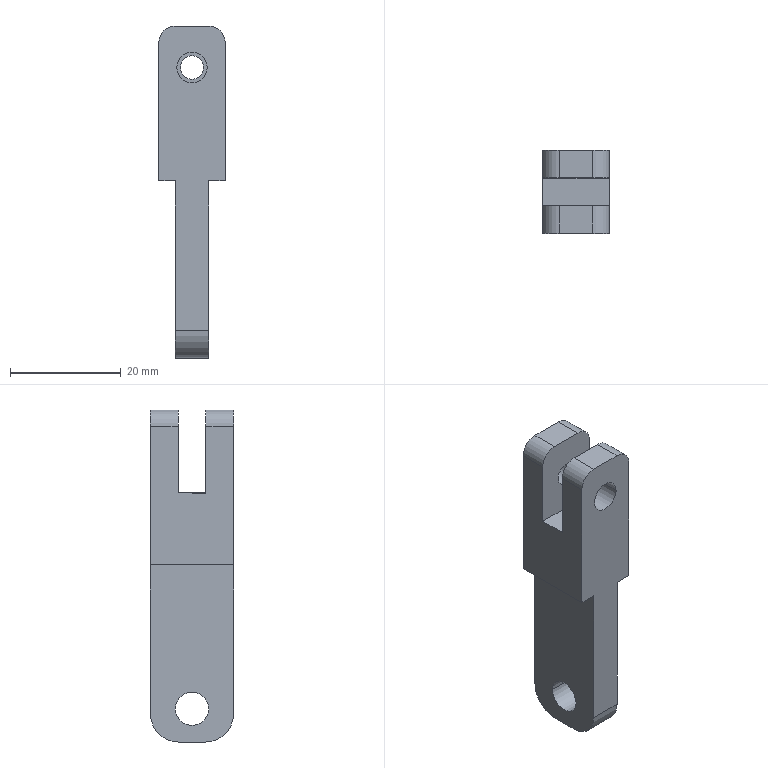Component | SolidWorks | ConnectingHinge1-2 | 1 solid | 26 faces | box 12 x 15 x 60 mm | volume 6559 mm3 | plane 14 | cylinder 12 | commonest cylinder face diameters 6 x6 4.2 x2 5.5 x2 10 x2
build123d program:
from build123d import *

# Parameters (mm, degrees)
SKETCH1_W           = 12
SKETCH1_H           = 60
BOSS_EXTRUDE1_DEPTH = 15
SKETCH2_W           = 5
SKETCH2_H           = 15
CUT_EXTRUDE1_DEPTH  = 64
CUT_EXTRUDE2_REACH  = 65
SKETCH3_R           = 2.75
M5_TAPPED_HOLE1_D   = 4.2
SKETCH6_R           = 3
CUT_EXTRUDE3_DEPTH  = 64
SKETCH7_W           = 3
SKETCH7_H           = 32
CUT_EXTRUDE4_DEPTH  = 64
FILLET1_R           = 5
FILLET2_R           = 3


with BuildPart() as part:
    # Sketch1 → Boss-Extrude1 (new body)
    with BuildSketch(Plane.XY):
        with Locations((6, 30)):
            Rectangle(SKETCH1_W, SKETCH1_H)
    extrude(amount=BOSS_EXTRUDE1_DEPTH)

    # Sketch2 → Cut-Extrude1 (cut, through all)
    with BuildSketch(Plane(origin=(12, 0, 0), x_dir=(0, 0, -1), z_dir=(1, 0, 0))):
        with Locations((-7.5, 7.5)):
            Rectangle(SKETCH2_W, SKETCH2_H)
    extrude(amount=-CUT_EXTRUDE1_DEPTH, mode=Mode.SUBTRACT)

    # Sketch3 → Cut-Extrude2 (cut, up to next)
    with BuildSketch(Plane(origin=(0, 0, 0), x_dir=(-1, 0, 0), z_dir=(0, 0, -1)), mode=Mode.PRIVATE) as cut_extrude2_sk1:
        with Locations((-6, 7.5)):
            Circle(SKETCH3_R)
    cut_extrude2_tool1 = extrude(cut_extrude2_sk1.sketch, amount=-CUT_EXTRUDE2_REACH, mode=Mode.PRIVATE) & part.part
    add(cut_extrude2_tool1.solids().sort_by_distance((6, 7.5, 0))[0], mode=Mode.SUBTRACT)

    # M5 Tapped Hole1 (through all)
    with Locations(Plane(origin=(6, 7.5, 15), x_dir=(1, 0, 0), z_dir=(0, 0, 1))):
        with Locations((0, 0)):
            Hole(M5_TAPPED_HOLE1_D / 2)

    # Sketch6 → Cut-Extrude3 (cut, through all)
    with BuildSketch(Plane.ZY):
        with Locations((7.5, 54)):
            Circle(SKETCH6_R)
    extrude(amount=-CUT_EXTRUDE3_DEPTH, mode=Mode.SUBTRACT)

    # Sketch7 → Cut-Extrude4 (cut, through all)
    with BuildSketch(Plane.XY.offset(15)):
        with Locations((1.5, 44)):
            Rectangle(SKETCH7_W, SKETCH7_H)
        with Locations((10.5, 44)):
            Rectangle(SKETCH7_W, SKETCH7_H)
    extrude(amount=-CUT_EXTRUDE4_DEPTH, mode=Mode.SUBTRACT)

    # Fillet1
    fillet1_edges = [part.edges().sort_by_distance(p)[0] for p in [
        (6, 60, 0),
        (6, 60, 15),
    ]]
    fillet(fillet1_edges, radius=FILLET1_R)

    # Fillet2
    fillet2_edges = [part.edges().sort_by_distance(p)[0] for p in [
        (12, 0, 2.5),
        (0, 0, 2.5),
        (12, 0, 12.5),
        (0, 0, 12.5),
    ]]
    fillet(fillet2_edges, radius=FILLET2_R)


solid = part.part

# Placed as in the assembly
solid = solid.moved(Location((-16, -226.728, 142.5), (-90, 0, 0)))
STEP:
#1=COLOUR_RGB('',0.7922,0.8196,0.9333);
#2=FILL_AREA_STYLE_COLOUR('',#1);
#3=FILL_AREA_STYLE('',(#2));
#4=SURFACE_STYLE_FILL_AREA(#3);
#5=SURFACE_SIDE_STYLE('',(#4));
#6=SURFACE_STYLE_USAGE(.BOTH.,#5);
#7=PRESENTATION_STYLE_ASSIGNMENT((#6));
#8=CARTESIAN_POINT('',(-0.2756,-8.513,3.484));
#9=VERTEX_POINT('',#8);
#10=CARTESIAN_POINT('',(-0.2756,-8.749,3.484));
#11=VERTEX_POINT('',#10);
#12=CARTESIAN_POINT('',(-0.2756,-8.631,3.484));
#13=DIRECTION('',(1.,0.,0.));
#14=DIRECTION('',(-0.,0.,1.));
#15=AXIS2_PLACEMENT_3D('',#12,#13,#14);
#16=CIRCLE('',#15,0.1181);
#17=EDGE_CURVE('',#9,#11,#16,.T.);
#18=ORIENTED_EDGE('',*,*,#17,.T.);
#19=CARTESIAN_POINT('',(-0.5118,-8.749,3.484));
#20=VERTEX_POINT('',#19);
#21=CARTESIAN_POINT('',(-0.1575,-8.749,3.484));
#22=DIRECTION('',(-1.,-0.,-0.));
#23=VECTOR('',#22,39.37);
#24=LINE('',#21,#23);
#25=EDGE_CURVE('',#11,#20,#24,.T.);
#26=ORIENTED_EDGE('',*,*,#25,.T.);
#27=CARTESIAN_POINT('',(-0.5118,-8.513,3.484));
#28=VERTEX_POINT('',#27);
#29=CARTESIAN_POINT('',(-0.5118,-8.631,3.484));
#30=DIRECTION('',(-1.,-0.,-0.));
#31=DIRECTION('',(0.,0.,-1.));
#32=AXIS2_PLACEMENT_3D('',#29,#30,#31);
#33=CIRCLE('',#32,0.1181);
#34=EDGE_CURVE('',#20,#28,#33,.T.);
#35=ORIENTED_EDGE('',*,*,#34,.T.);
#36=CARTESIAN_POINT('',(-0.1575,-8.513,3.484));
#37=DIRECTION('',(-1.,-0.,-0.));
#38=VECTOR('',#37,39.37);
#39=LINE('',#36,#38);
#40=EDGE_CURVE('',#9,#28,#39,.T.);
#41=ORIENTED_EDGE('',*,*,#40,.F.);
#42=EDGE_LOOP('',(#18,#26,#35,#41));
#43=FACE_OUTER_BOUND('',#42,.T.);
#44=CARTESIAN_POINT('',(-0.1575,-8.631,3.484));
#45=DIRECTION('',(-1.,-0.,-0.));
#46=DIRECTION('',(-0.,1.,0.));
#47=AXIS2_PLACEMENT_3D('',#44,#45,#46);
#48=CYLINDRICAL_SURFACE('',#47,0.1181);
#49=ADVANCED_FACE('',(#43),#48,.F.);
#50=CARTESIAN_POINT('',(-0.4764,-8.533,5.315));
#51=VERTEX_POINT('',#50);
#52=CARTESIAN_POINT('',(-0.311,-8.533,5.315));
#53=VERTEX_POINT('',#52);
#54=CARTESIAN_POINT('',(-0.3937,-8.533,5.315));
#55=DIRECTION('',(-0.,1.,0.));
#56=DIRECTION('',(-0.,0.,1.));
#57=AXIS2_PLACEMENT_3D('',#54,#55,#56);
#58=CIRCLE('',#57,0.08268);
#59=EDGE_CURVE('',#51,#53,#58,.T.);
#60=ORIENTED_EDGE('',*,*,#59,.F.);
#61=CARTESIAN_POINT('',(-0.4764,-8.336,5.315));
#62=VERTEX_POINT('',#61);
#63=CARTESIAN_POINT('',(-0.4764,-8.336,5.315));
#64=DIRECTION('',(-0.,1.,0.));
#65=VECTOR('',#64,39.37);
#66=LINE('',#63,#65);
#67=EDGE_CURVE('',#51,#62,#66,.T.);
#68=ORIENTED_EDGE('',*,*,#67,.T.);
#69=CARTESIAN_POINT('',(-0.311,-8.336,5.315));
#70=VERTEX_POINT('',#69);
#71=CARTESIAN_POINT('',(-0.3937,-8.336,5.315));
#72=DIRECTION('',(-0.,1.,0.));
#73=DIRECTION('',(1.,0.,0.));
#74=AXIS2_PLACEMENT_3D('',#71,#72,#73);
#75=CIRCLE('',#74,0.08268);
#76=EDGE_CURVE('',#62,#70,#75,.T.);
#77=ORIENTED_EDGE('',*,*,#76,.T.);
#78=CARTESIAN_POINT('',(-0.311,-8.336,5.315));
#79=DIRECTION('',(-0.,1.,0.));
#80=VECTOR('',#79,39.37);
#81=LINE('',#78,#80);
#82=EDGE_CURVE('',#53,#70,#81,.T.);
#83=ORIENTED_EDGE('',*,*,#82,.F.);
#84=EDGE_LOOP('',(#60,#68,#77,#83));
#85=FACE_OUTER_BOUND('',#84,.T.);
#86=CARTESIAN_POINT('',(-0.3937,-8.336,5.315));
#87=DIRECTION('',(-0.,1.,0.));
#88=DIRECTION('',(1.,0.,0.));
#89=AXIS2_PLACEMENT_3D('',#86,#87,#88);
#90=CYLINDRICAL_SURFACE('',#89,0.08268);
#91=ADVANCED_FACE('',(#85),#90,.F.);
#92=CARTESIAN_POINT('',(-0.502,-8.729,5.315));
#93=VERTEX_POINT('',#92);
#94=CARTESIAN_POINT('',(-0.2854,-8.729,5.315));
#95=VERTEX_POINT('',#94);
#96=CARTESIAN_POINT('',(-0.3937,-8.729,5.315));
#97=DIRECTION('',(-0.,1.,0.));
#98=DIRECTION('',(0.,0.,-1.));
#99=AXIS2_PLACEMENT_3D('',#96,#97,#98);
#100=CIRCLE('',#99,0.1083);
#101=EDGE_CURVE('',#93,#95,#100,.T.);
#102=ORIENTED_EDGE('',*,*,#101,.T.);
#103=CARTESIAN_POINT('',(-0.2854,-8.926,5.315));
#104=VERTEX_POINT('',#103);
#105=CARTESIAN_POINT('',(-0.2854,-8.336,5.315));
#106=DIRECTION('',(0.,-1.,-0.));
#107=VECTOR('',#106,39.37);
#108=LINE('',#105,#107);
#109=EDGE_CURVE('',#95,#104,#108,.T.);
#110=ORIENTED_EDGE('',*,*,#109,.T.);
#111=CARTESIAN_POINT('',(-0.502,-8.926,5.315));
#112=VERTEX_POINT('',#111);
#113=CARTESIAN_POINT('',(-0.3937,-8.926,5.315));
#114=DIRECTION('',(0.,-1.,-0.));
#115=DIRECTION('',(-1.,0.,0.));
#116=AXIS2_PLACEMENT_3D('',#113,#114,#115);
#117=CIRCLE('',#116,0.1083);
#118=EDGE_CURVE('',#104,#112,#117,.T.);
#119=ORIENTED_EDGE('',*,*,#118,.T.);
#120=CARTESIAN_POINT('',(-0.502,-8.336,5.315));
#121=DIRECTION('',(0.,-1.,-0.));
#122=VECTOR('',#121,39.37);
#123=LINE('',#120,#122);
#124=EDGE_CURVE('',#93,#112,#123,.T.);
#125=ORIENTED_EDGE('',*,*,#124,.F.);
#126=EDGE_LOOP('',(#102,#110,#119,#125));
#127=FACE_OUTER_BOUND('',#126,.T.);
#128=CARTESIAN_POINT('',(-0.3937,-8.336,5.315));
#129=DIRECTION('',(0.,-1.,-0.));
#130=DIRECTION('',(-1.,0.,0.));
#131=AXIS2_PLACEMENT_3D('',#128,#129,#130);
#132=CYLINDRICAL_SURFACE('',#131,0.1083);
#133=ADVANCED_FACE('',(#127),#132,.F.);
#134=CARTESIAN_POINT('',(-0.6299,-8.336,4.508));
#135=VERTEX_POINT('',#134);
#136=CARTESIAN_POINT('',(-0.6299,-8.336,5.492));
#137=VERTEX_POINT('',#136);
#138=CARTESIAN_POINT('',(-0.6299,-8.336,5.61));
#139=DIRECTION('',(-0.,-0.,1.));
#140=VECTOR('',#139,39.37);
#141=LINE('',#138,#140);
#142=EDGE_CURVE('',#135,#137,#141,.T.);
#143=ORIENTED_EDGE('',*,*,#142,.T.);
#144=CARTESIAN_POINT('',(-0.5118,-8.336,5.61));
#145=VERTEX_POINT('',#144);
#146=CARTESIAN_POINT('',(-0.5118,-8.336,5.492));
#147=DIRECTION('',(-0.,1.,0.));
#148=DIRECTION('',(-1.,0.,0.));
#149=AXIS2_PLACEMENT_3D('',#146,#147,#148);
#150=CIRCLE('',#149,0.1181);
#151=EDGE_CURVE('',#137,#145,#150,.T.);
#152=ORIENTED_EDGE('',*,*,#151,.T.);
#153=CARTESIAN_POINT('',(-0.2756,-8.336,5.61));
#154=VERTEX_POINT('',#153);
#155=CARTESIAN_POINT('',(-0.6299,-8.336,5.61));
#156=DIRECTION('',(1.,0.,0.));
#157=VECTOR('',#156,39.37);
#158=LINE('',#155,#157);
#159=EDGE_CURVE('',#145,#154,#158,.T.);
#160=ORIENTED_EDGE('',*,*,#159,.T.);
#161=CARTESIAN_POINT('',(-0.1575,-8.336,5.492));
#162=VERTEX_POINT('',#161);
#163=CARTESIAN_POINT('',(-0.2756,-8.336,5.492));
#164=DIRECTION('',(-0.,1.,0.));
#165=DIRECTION('',(-1.,0.,0.));
#166=AXIS2_PLACEMENT_3D('',#163,#164,#165);
#167=CIRCLE('',#166,0.1181);
#168=EDGE_CURVE('',#154,#162,#167,.T.);
#169=ORIENTED_EDGE('',*,*,#168,.T.);
#170=CARTESIAN_POINT('',(-0.1575,-8.336,4.508));
#171=VERTEX_POINT('',#170);
#172=CARTESIAN_POINT('',(-0.1575,-8.336,5.61));
#173=DIRECTION('',(0.,0.,-1.));
#174=VECTOR('',#173,39.37);
#175=LINE('',#172,#174);
#176=EDGE_CURVE('',#162,#171,#175,.T.);
#177=ORIENTED_EDGE('',*,*,#176,.T.);
#178=CARTESIAN_POINT('',(-0.2756,-8.336,4.508));
#179=VERTEX_POINT('',#178);
#180=CARTESIAN_POINT('',(-0.1575,-8.336,4.508));
#181=DIRECTION('',(1.,0.,0.));
#182=VECTOR('',#181,39.37);
#183=LINE('',#180,#182);
#184=EDGE_CURVE('',#179,#171,#183,.T.);
#185=ORIENTED_EDGE('',*,*,#184,.F.);
#186=CARTESIAN_POINT('',(-0.2756,-8.336,3.445));
#187=VERTEX_POINT('',#186);
#188=CARTESIAN_POINT('',(-0.2756,-8.336,3.248));
#189=DIRECTION('',(-0.,-0.,1.));
#190=VECTOR('',#189,39.37);
#191=LINE('',#188,#190);
#192=EDGE_CURVE('',#187,#179,#191,.T.);
#193=ORIENTED_EDGE('',*,*,#192,.F.);
#194=CARTESIAN_POINT('',(-0.5118,-8.336,3.445));
#195=VERTEX_POINT('',#194);
#196=CARTESIAN_POINT('',(-0.6299,-8.336,3.445));
#197=DIRECTION('',(-1.,-0.,-0.));
#198=VECTOR('',#197,39.37);
#199=LINE('',#196,#198);
#200=EDGE_CURVE('',#187,#195,#199,.T.);
#201=ORIENTED_EDGE('',*,*,#200,.T.);
#202=CARTESIAN_POINT('',(-0.5118,-8.336,4.508));
#203=VERTEX_POINT('',#202);
#204=CARTESIAN_POINT('',(-0.5118,-8.336,3.248));
#205=DIRECTION('',(0.,0.,-1.));
#206=VECTOR('',#205,39.37);
#207=LINE('',#204,#206);
#208=EDGE_CURVE('',#203,#195,#207,.T.);
#209=ORIENTED_EDGE('',*,*,#208,.F.);
#210=CARTESIAN_POINT('',(-0.6299,-8.336,4.508));
#211=DIRECTION('',(1.,0.,0.));
#212=VECTOR('',#211,39.37);
#213=LINE('',#210,#212);
#214=EDGE_CURVE('',#135,#203,#213,.T.);
#215=ORIENTED_EDGE('',*,*,#214,.F.);
#216=EDGE_LOOP('',(#143,#152,#160,#169,#177,#185,#193,#201,#209,#215));
#217=FACE_OUTER_BOUND('',#216,.T.);
#218=CARTESIAN_POINT('',(-0.3937,-8.336,5.315));
#219=DIRECTION('',(-0.,1.,0.));
#220=DIRECTION('',(1.,0.,0.));
#221=AXIS2_PLACEMENT_3D('',#218,#219,#220);
#222=CIRCLE('',#221,0.08268);
#223=EDGE_CURVE('',#70,#62,#222,.T.);
#224=ORIENTED_EDGE('',*,*,#223,.F.);
#225=ORIENTED_EDGE('',*,*,#76,.F.);
#226=EDGE_LOOP('',(#224,#225));
#227=FACE_BOUND('',#226,.T.);
#228=CARTESIAN_POINT('',(-0.6299,-8.336,5.61));
#229=DIRECTION('',(0.,-1.,-0.));
#230=DIRECTION('',(-1.,-0.,-0.));
#231=AXIS2_PLACEMENT_3D('',#228,#229,#230);
#232=PLANE('',#231);
#233=ADVANCED_FACE('',(#217,#227),#232,.F.);
#234=ORIENTED_EDGE('',*,*,#159,.F.);
#235=CARTESIAN_POINT('',(-0.5118,-8.533,5.61));
#236=VERTEX_POINT('',#235);
#237=CARTESIAN_POINT('',(-0.5118,-8.336,5.61));
#238=DIRECTION('',(0.,-1.,-0.));
#239=VECTOR('',#238,39.37);
#240=LINE('',#237,#239);
#241=EDGE_CURVE('',#145,#236,#240,.T.);
#242=ORIENTED_EDGE('',*,*,#241,.T.);
#243=CARTESIAN_POINT('',(-0.2756,-8.533,5.61));
#244=VERTEX_POINT('',#243);
#245=CARTESIAN_POINT('',(-0.6299,-8.533,5.61));
#246=DIRECTION('',(1.,0.,0.));
#247=VECTOR('',#246,39.37);
#248=LINE('',#245,#247);
#249=EDGE_CURVE('',#236,#244,#248,.T.);
#250=ORIENTED_EDGE('',*,*,#249,.T.);
#251=CARTESIAN_POINT('',(-0.2756,-8.336,5.61));
#252=DIRECTION('',(-0.,1.,0.));
#253=VECTOR('',#252,39.37);
#254=LINE('',#251,#253);
#255=EDGE_CURVE('',#244,#154,#254,.T.);
#256=ORIENTED_EDGE('',*,*,#255,.T.);
#257=EDGE_LOOP('',(#234,#242,#250,#256));
#258=FACE_OUTER_BOUND('',#257,.T.);
#259=CARTESIAN_POINT('',(-0.6299,-8.336,5.61));
#260=DIRECTION('',(0.,0.,-1.));
#261=DIRECTION('',(-0.,1.,0.));
#262=AXIS2_PLACEMENT_3D('',#259,#260,#261);
#263=PLANE('',#262);
#264=ADVANCED_FACE('',(#258),#263,.F.);
#265=CARTESIAN_POINT('',(-0.6299,-8.533,5.02));
#266=VERTEX_POINT('',#265);
#267=CARTESIAN_POINT('',(-0.6299,-8.533,5.492));
#268=VERTEX_POINT('',#267);
#269=CARTESIAN_POINT('',(-0.6299,-8.533,5.02));
#270=DIRECTION('',(-0.,-0.,1.));
#271=VECTOR('',#270,39.37);
#272=LINE('',#269,#271);
#273=EDGE_CURVE('',#266,#268,#272,.T.);
#274=ORIENTED_EDGE('',*,*,#273,.T.);
#275=CARTESIAN_POINT('',(-0.6299,-8.336,5.492));
#276=DIRECTION('',(-0.,1.,0.));
#277=VECTOR('',#276,39.37);
#278=LINE('',#275,#277);
#279=EDGE_CURVE('',#268,#137,#278,.T.);
#280=ORIENTED_EDGE('',*,*,#279,.T.);
#281=ORIENTED_EDGE('',*,*,#142,.F.);
#282=CARTESIAN_POINT('',(-0.6299,-8.926,4.508));
#283=VERTEX_POINT('',#282);
#284=CARTESIAN_POINT('',(-0.6299,-8.926,4.508));
#285=DIRECTION('',(-0.,1.,0.));
#286=VECTOR('',#285,39.37);
#287=LINE('',#284,#286);
#288=EDGE_CURVE('',#283,#135,#287,.T.);
#289=ORIENTED_EDGE('',*,*,#288,.F.);
#290=CARTESIAN_POINT('',(-0.6299,-8.926,5.492));
#291=VERTEX_POINT('',#290);
#292=CARTESIAN_POINT('',(-0.6299,-8.926,5.61));
#293=DIRECTION('',(-0.,-0.,1.));
#294=VECTOR('',#293,39.37);
#295=LINE('',#292,#294);
#296=EDGE_CURVE('',#283,#291,#295,.T.);
#297=ORIENTED_EDGE('',*,*,#296,.T.);
#298=CARTESIAN_POINT('',(-0.6299,-8.729,5.492));
#299=VERTEX_POINT('',#298);
#300=CARTESIAN_POINT('',(-0.6299,-8.336,5.492));
#301=DIRECTION('',(-0.,1.,0.));
#302=VECTOR('',#301,39.37);
#303=LINE('',#300,#302);
#304=EDGE_CURVE('',#291,#299,#303,.T.);
#305=ORIENTED_EDGE('',*,*,#304,.T.);
#306=CARTESIAN_POINT('',(-0.6299,-8.729,5.02));
#307=VERTEX_POINT('',#306);
#308=CARTESIAN_POINT('',(-0.6299,-8.729,5.02));
#309=DIRECTION('',(0.,0.,-1.));
#310=VECTOR('',#309,39.37);
#311=LINE('',#308,#310);
#312=EDGE_CURVE('',#299,#307,#311,.T.);
#313=ORIENTED_EDGE('',*,*,#312,.T.);
#314=CARTESIAN_POINT('',(-0.6299,-8.533,5.02));
#315=DIRECTION('',(-0.,1.,0.));
#316=VECTOR('',#315,39.37);
#317=LINE('',#314,#316);
#318=EDGE_CURVE('',#307,#266,#317,.T.);
#319=ORIENTED_EDGE('',*,*,#318,.T.);
#320=EDGE_LOOP('',(#274,#280,#281,#289,#297,#305,#313,#319));
#321=FACE_OUTER_BOUND('',#320,.T.);
#322=CARTESIAN_POINT('',(-0.6299,-8.336,5.61));
#323=DIRECTION('',(1.,0.,0.));
#324=DIRECTION('',(0.,-1.,-0.));
#325=AXIS2_PLACEMENT_3D('',#322,#323,#324);
#326=PLANE('',#325);
#327=ADVANCED_FACE('',(#321),#326,.F.);
#328=CARTESIAN_POINT('',(-0.5118,-8.729,5.61));
#329=VERTEX_POINT('',#328);
#330=CARTESIAN_POINT('',(-0.2756,-8.729,5.61));
#331=VERTEX_POINT('',#330);
#332=CARTESIAN_POINT('',(-0.6299,-8.729,5.61));
#333=DIRECTION('',(1.,0.,0.));
#334=VECTOR('',#333,39.37);
#335=LINE('',#332,#334);
#336=EDGE_CURVE('',#329,#331,#335,.T.);
#337=ORIENTED_EDGE('',*,*,#336,.F.);
#338=CARTESIAN_POINT('',(-0.5118,-8.926,5.61));
#339=VERTEX_POINT('',#338);
#340=CARTESIAN_POINT('',(-0.5118,-8.336,5.61));
#341=DIRECTION('',(0.,-1.,-0.));
#342=VECTOR('',#341,39.37);
#343=LINE('',#340,#342);
#344=EDGE_CURVE('',#329,#339,#343,.T.);
#345=ORIENTED_EDGE('',*,*,#344,.T.);
#346=CARTESIAN_POINT('',(-0.2756,-8.926,5.61));
#347=VERTEX_POINT('',#346);
#348=CARTESIAN_POINT('',(-0.6299,-8.926,5.61));
#349=DIRECTION('',(1.,0.,0.));
#350=VECTOR('',#349,39.37);
#351=LINE('',#348,#350);
#352=EDGE_CURVE('',#339,#347,#351,.T.);
#353=ORIENTED_EDGE('',*,*,#352,.T.);
#354=CARTESIAN_POINT('',(-0.2756,-8.336,5.61));
#355=DIRECTION('',(-0.,1.,0.));
#356=VECTOR('',#355,39.37);
#357=LINE('',#354,#356);
#358=EDGE_CURVE('',#347,#331,#357,.T.);
#359=ORIENTED_EDGE('',*,*,#358,.T.);
#360=EDGE_LOOP('',(#337,#345,#353,#359));
#361=FACE_OUTER_BOUND('',#360,.T.);
#362=CARTESIAN_POINT('',(-0.6299,-8.336,5.61));
#363=DIRECTION('',(0.,0.,-1.));
#364=DIRECTION('',(-0.,1.,0.));
#365=AXIS2_PLACEMENT_3D('',#362,#363,#364);
#366=PLANE('',#365);
#367=ADVANCED_FACE('',(#361),#366,.F.);
#368=ORIENTED_EDGE('',*,*,#176,.F.);
#369=CARTESIAN_POINT('',(-0.1575,-8.533,5.492));
#370=VERTEX_POINT('',#369);
#371=CARTESIAN_POINT('',(-0.1575,-8.336,5.492));
#372=DIRECTION('',(0.,-1.,-0.));
#373=VECTOR('',#372,39.37);
#374=LINE('',#371,#373);
#375=EDGE_CURVE('',#162,#370,#374,.T.);
#376=ORIENTED_EDGE('',*,*,#375,.T.);
#377=CARTESIAN_POINT('',(-0.1575,-8.533,5.02));
#378=VERTEX_POINT('',#377);
#379=CARTESIAN_POINT('',(-0.1575,-8.533,5.02));
#380=DIRECTION('',(-0.,-0.,1.));
#381=VECTOR('',#380,39.37);
#382=LINE('',#379,#381);
#383=EDGE_CURVE('',#378,#370,#382,.T.);
#384=ORIENTED_EDGE('',*,*,#383,.F.);
#385=CARTESIAN_POINT('',(-0.1575,-8.729,5.02));
#386=VERTEX_POINT('',#385);
#387=CARTESIAN_POINT('',(-0.1575,-8.533,5.02));
#388=DIRECTION('',(-0.,1.,0.));
#389=VECTOR('',#388,39.37);
#390=LINE('',#387,#389);
#391=EDGE_CURVE('',#386,#378,#390,.T.);
#392=ORIENTED_EDGE('',*,*,#391,.F.);
#393=CARTESIAN_POINT('',(-0.1575,-8.729,5.492));
#394=VERTEX_POINT('',#393);
#395=CARTESIAN_POINT('',(-0.1575,-8.729,5.02));
#396=DIRECTION('',(0.,0.,-1.));
#397=VECTOR('',#396,39.37);
#398=LINE('',#395,#397);
#399=EDGE_CURVE('',#394,#386,#398,.T.);
#400=ORIENTED_EDGE('',*,*,#399,.F.);
#401=CARTESIAN_POINT('',(-0.1575,-8.926,5.492));
#402=VERTEX_POINT('',#401);
#403=CARTESIAN_POINT('',(-0.1575,-8.336,5.492));
#404=DIRECTION('',(0.,-1.,-0.));
#405=VECTOR('',#404,39.37);
#406=LINE('',#403,#405);
#407=EDGE_CURVE('',#394,#402,#406,.T.);
#408=ORIENTED_EDGE('',*,*,#407,.T.);
#409=CARTESIAN_POINT('',(-0.1575,-8.926,4.508));
#410=VERTEX_POINT('',#409);
#411=CARTESIAN_POINT('',(-0.1575,-8.926,5.61));
#412=DIRECTION('',(0.,0.,-1.));
#413=VECTOR('',#412,39.37);
#414=LINE('',#411,#413);
#415=EDGE_CURVE('',#402,#410,#414,.T.);
#416=ORIENTED_EDGE('',*,*,#415,.T.);
#417=CARTESIAN_POINT('',(-0.1575,-8.926,4.508));
#418=DIRECTION('',(-0.,1.,0.));
#419=VECTOR('',#418,39.37);
#420=LINE('',#417,#419);
#421=EDGE_CURVE('',#410,#171,#420,.T.);
#422=ORIENTED_EDGE('',*,*,#421,.T.);
#423=EDGE_LOOP('',(#368,#376,#384,#392,#400,#408,#416,#422));
#424=FACE_OUTER_BOUND('',#423,.T.);
#425=CARTESIAN_POINT('',(-0.1575,-8.336,5.61));
#426=DIRECTION('',(-1.,-0.,-0.));
#427=DIRECTION('',(-0.,1.,0.));
#428=AXIS2_PLACEMENT_3D('',#425,#426,#427);
#429=PLANE('',#428);
#430=ADVANCED_FACE('',(#424),#429,.F.);
#431=CARTESIAN_POINT('',(-0.5118,-8.729,3.248));
#432=VERTEX_POINT('',#431);
#433=CARTESIAN_POINT('',(-0.5118,-8.533,3.248));
#434=VERTEX_POINT('',#433);
#435=CARTESIAN_POINT('',(-0.5118,-8.926,3.248));
#436=DIRECTION('',(-0.,1.,0.));
#437=VECTOR('',#436,39.37);
#438=LINE('',#435,#437);
#439=EDGE_CURVE('',#432,#434,#438,.T.);
#440=ORIENTED_EDGE('',*,*,#439,.T.);
#441=CARTESIAN_POINT('',(-0.2756,-8.533,3.248));
#442=VERTEX_POINT('',#441);
#443=CARTESIAN_POINT('',(-0.6299,-8.533,3.248));
#444=DIRECTION('',(1.,0.,0.));
#445=VECTOR('',#444,39.37);
#446=LINE('',#443,#445);
#447=EDGE_CURVE('',#434,#442,#446,.T.);
#448=ORIENTED_EDGE('',*,*,#447,.T.);
#449=CARTESIAN_POINT('',(-0.2756,-8.729,3.248));
#450=VERTEX_POINT('',#449);
#451=CARTESIAN_POINT('',(-0.2756,-8.926,3.248));
#452=DIRECTION('',(-0.,1.,0.));
#453=VECTOR('',#452,39.37);
#454=LINE('',#451,#453);
#455=EDGE_CURVE('',#450,#442,#454,.T.);
#456=ORIENTED_EDGE('',*,*,#455,.F.);
#457=CARTESIAN_POINT('',(-0.5118,-8.729,3.248));
#458=DIRECTION('',(-1.,-0.,-0.));
#459=VECTOR('',#458,39.37);
#460=LINE('',#457,#459);
#461=EDGE_CURVE('',#450,#432,#460,.T.);
#462=ORIENTED_EDGE('',*,*,#461,.T.);
#463=EDGE_LOOP('',(#440,#448,#456,#462));
#464=FACE_OUTER_BOUND('',#463,.T.);
#465=CARTESIAN_POINT('',(-0.6299,-8.336,3.248));
#466=DIRECTION('',(-0.,-0.,1.));
#467=DIRECTION('',(0.,-1.,-0.));
#468=AXIS2_PLACEMENT_3D('',#465,#466,#467);
#469=PLANE('',#468);
#470=ADVANCED_FACE('',(#464),#469,.F.);
#471=ORIENTED_EDGE('',*,*,#352,.F.);
#472=CARTESIAN_POINT('',(-0.5118,-8.926,5.492));
#473=DIRECTION('',(0.,-1.,-0.));
#474=DIRECTION('',(-1.,0.,0.));
#475=AXIS2_PLACEMENT_3D('',#472,#473,#474);
#476=CIRCLE('',#475,0.1181);
#477=EDGE_CURVE('',#339,#291,#476,.T.);
#478=ORIENTED_EDGE('',*,*,#477,.T.);
#479=ORIENTED_EDGE('',*,*,#296,.F.);
#480=CARTESIAN_POINT('',(-0.5118,-8.926,4.508));
#481=VERTEX_POINT('',#480);
#482=CARTESIAN_POINT('',(-0.6299,-8.926,4.508));
#483=DIRECTION('',(1.,0.,0.));
#484=VECTOR('',#483,39.37);
#485=LINE('',#482,#484);
#486=EDGE_CURVE('',#283,#481,#485,.T.);
#487=ORIENTED_EDGE('',*,*,#486,.T.);
#488=CARTESIAN_POINT('',(-0.5118,-8.926,3.445));
#489=VERTEX_POINT('',#488);
#490=CARTESIAN_POINT('',(-0.5118,-8.926,3.248));
#491=DIRECTION('',(0.,0.,-1.));
#492=VECTOR('',#491,39.37);
#493=LINE('',#490,#492);
#494=EDGE_CURVE('',#481,#489,#493,.T.);
#495=ORIENTED_EDGE('',*,*,#494,.T.);
#496=CARTESIAN_POINT('',(-0.2756,-8.926,3.445));
#497=VERTEX_POINT('',#496);
#498=CARTESIAN_POINT('',(-0.2756,-8.926,3.445));
#499=DIRECTION('',(1.,0.,0.));
#500=VECTOR('',#499,39.37);
#501=LINE('',#498,#500);
#502=EDGE_CURVE('',#489,#497,#501,.T.);
#503=ORIENTED_EDGE('',*,*,#502,.T.);
#504=CARTESIAN_POINT('',(-0.2756,-8.926,4.508));
#505=VERTEX_POINT('',#504);
#506=CARTESIAN_POINT('',(-0.2756,-8.926,3.248));
#507=DIRECTION('',(-0.,-0.,1.));
#508=VECTOR('',#507,39.37);
#509=LINE('',#506,#508);
#510=EDGE_CURVE('',#497,#505,#509,.T.);
#511=ORIENTED_EDGE('',*,*,#510,.T.);
#512=CARTESIAN_POINT('',(-0.1575,-8.926,4.508));
#513=DIRECTION('',(1.,0.,0.));
#514=VECTOR('',#513,39.37);
#515=LINE('',#512,#514);
#516=EDGE_CURVE('',#505,#410,#515,.T.);
#517=ORIENTED_EDGE('',*,*,#516,.T.);
#518=ORIENTED_EDGE('',*,*,#415,.F.);
#519=CARTESIAN_POINT('',(-0.2756,-8.926,5.492));
#520=DIRECTION('',(0.,-1.,-0.));
#521=DIRECTION('',(-1.,0.,0.));
#522=AXIS2_PLACEMENT_3D('',#519,#520,#521);
#523=CIRCLE('',#522,0.1181);
#524=EDGE_CURVE('',#402,#347,#523,.T.);
#525=ORIENTED_EDGE('',*,*,#524,.T.);
#526=EDGE_LOOP('',(#471,#478,#479,#487,#495,#503,#511,#517,#518,#525));
#527=FACE_OUTER_BOUND('',#526,.T.);
#528=CARTESIAN_POINT('',(-0.3937,-8.926,5.315));
#529=DIRECTION('',(0.,-1.,-0.));
#530=DIRECTION('',(-1.,0.,0.));
#531=AXIS2_PLACEMENT_3D('',#528,#529,#530);
#532=CIRCLE('',#531,0.1083);
#533=EDGE_CURVE('',#112,#104,#532,.T.);
#534=ORIENTED_EDGE('',*,*,#533,.F.);
#535=ORIENTED_EDGE('',*,*,#118,.F.);
#536=EDGE_LOOP('',(#534,#535));
#537=FACE_BOUND('',#536,.T.);
#538=CARTESIAN_POINT('',(-0.6299,-8.926,5.61));
#539=DIRECTION('',(0.,-1.,-0.));
#540=DIRECTION('',(-1.,-0.,-0.));
#541=AXIS2_PLACEMENT_3D('',#538,#539,#540);
#542=PLANE('',#541);
#543=ADVANCED_FACE('',(#527,#537),#542,.T.);
#544=CARTESIAN_POINT('',(-0.3937,-8.533,5.315));
#545=DIRECTION('',(-0.,1.,0.));
#546=DIRECTION('',(-0.,0.,1.));
#547=AXIS2_PLACEMENT_3D('',#544,#545,#546);
#548=CIRCLE('',#547,0.08268);
#549=EDGE_CURVE('',#53,#51,#548,.T.);
#550=ORIENTED_EDGE('',*,*,#549,.T.);
#551=ORIENTED_EDGE('',*,*,#59,.T.);
#552=EDGE_LOOP('',(#550,#551));
#553=FACE_BOUND('',#552,.T.);
#554=ORIENTED_EDGE('',*,*,#249,.F.);
#555=CARTESIAN_POINT('',(-0.5118,-8.533,5.492));
#556=DIRECTION('',(0.,-1.,-0.));
#557=DIRECTION('',(-0.,0.,1.));
#558=AXIS2_PLACEMENT_3D('',#555,#556,#557);
#559=CIRCLE('',#558,0.1181);
#560=EDGE_CURVE('',#236,#268,#559,.T.);
#561=ORIENTED_EDGE('',*,*,#560,.T.);
#562=ORIENTED_EDGE('',*,*,#273,.F.);
#563=CARTESIAN_POINT('',(-0.6299,-8.533,5.02));
#564=DIRECTION('',(1.,0.,0.));
#565=VECTOR('',#564,39.37);
#566=LINE('',#563,#565);
#567=EDGE_CURVE('',#266,#378,#566,.T.);
#568=ORIENTED_EDGE('',*,*,#567,.T.);
#569=ORIENTED_EDGE('',*,*,#383,.T.);
#570=CARTESIAN_POINT('',(-0.2756,-8.533,5.492));
#571=DIRECTION('',(0.,-1.,-0.));
#572=DIRECTION('',(0.,0.,1.));
#573=AXIS2_PLACEMENT_3D('',#570,#571,#572);
#574=CIRCLE('',#573,0.1181);
#575=EDGE_CURVE('',#370,#244,#574,.T.);
#576=ORIENTED_EDGE('',*,*,#575,.T.);
#577=EDGE_LOOP('',(#554,#561,#562,#568,#569,#576));
#578=FACE_OUTER_BOUND('',#577,.T.);
#579=CARTESIAN_POINT('',(-0.6299,-8.533,5.02));
#580=DIRECTION('',(-0.,1.,0.));
#581=DIRECTION('',(-0.,-0.,1.));
#582=AXIS2_PLACEMENT_3D('',#579,#580,#581);
#583=PLANE('',#582);
#584=ADVANCED_FACE('',(#553,#578),#583,.F.);
#585=ORIENTED_EDGE('',*,*,#391,.T.);
#586=ORIENTED_EDGE('',*,*,#567,.F.);
#587=ORIENTED_EDGE('',*,*,#318,.F.);
#588=CARTESIAN_POINT('',(-0.6299,-8.729,5.02));
#589=DIRECTION('',(1.,0.,0.));
#590=VECTOR('',#589,39.37);
#591=LINE('',#588,#590);
#592=EDGE_CURVE('',#307,#386,#591,.T.);
#593=ORIENTED_EDGE('',*,*,#592,.T.);
#594=EDGE_LOOP('',(#585,#586,#587,#593));
#595=FACE_OUTER_BOUND('',#594,.T.);
#596=CARTESIAN_POINT('',(-0.6299,-8.533,5.02));
#597=DIRECTION('',(0.,0.,-1.));
#598=DIRECTION('',(-0.,1.,0.));
#599=AXIS2_PLACEMENT_3D('',#596,#597,#598);
#600=PLANE('',#599);
#601=ADVANCED_FACE('',(#595),#600,.F.);
#602=ORIENTED_EDGE('',*,*,#101,.F.);
#603=CARTESIAN_POINT('',(-0.3937,-8.729,5.315));
#604=DIRECTION('',(-0.,1.,0.));
#605=DIRECTION('',(0.,0.,-1.));
#606=AXIS2_PLACEMENT_3D('',#603,#604,#605);
#607=CIRCLE('',#606,0.1083);
#608=EDGE_CURVE('',#95,#93,#607,.T.);
#609=ORIENTED_EDGE('',*,*,#608,.F.);
#610=EDGE_LOOP('',(#602,#609));
#611=FACE_BOUND('',#610,.T.);
#612=ORIENTED_EDGE('',*,*,#312,.F.);
#613=CARTESIAN_POINT('',(-0.5118,-8.729,5.492));
#614=DIRECTION('',(-0.,1.,0.));
#615=DIRECTION('',(0.,0.,-1.));
#616=AXIS2_PLACEMENT_3D('',#613,#614,#615);
#617=CIRCLE('',#616,0.1181);
#618=EDGE_CURVE('',#299,#329,#617,.T.);
#619=ORIENTED_EDGE('',*,*,#618,.T.);
#620=ORIENTED_EDGE('',*,*,#336,.T.);
#621=CARTESIAN_POINT('',(-0.2756,-8.729,5.492));
#622=DIRECTION('',(-0.,1.,0.));
#623=DIRECTION('',(0.,0.,-1.));
#624=AXIS2_PLACEMENT_3D('',#621,#622,#623);
#625=CIRCLE('',#624,0.1181);
#626=EDGE_CURVE('',#331,#394,#625,.T.);
#627=ORIENTED_EDGE('',*,*,#626,.T.);
#628=ORIENTED_EDGE('',*,*,#399,.T.);
#629=ORIENTED_EDGE('',*,*,#592,.F.);
#630=EDGE_LOOP('',(#612,#619,#620,#627,#628,#629));
#631=FACE_OUTER_BOUND('',#630,.T.);
#632=CARTESIAN_POINT('',(-0.6299,-8.729,5.02));
#633=DIRECTION('',(0.,-1.,-0.));
#634=DIRECTION('',(0.,0.,-1.));
#635=AXIS2_PLACEMENT_3D('',#632,#633,#634);
#636=PLANE('',#635);
#637=ADVANCED_FACE('',(#611,#631),#636,.F.);
#638=ORIENTED_EDGE('',*,*,#109,.F.);
#639=ORIENTED_EDGE('',*,*,#608,.T.);
#640=ORIENTED_EDGE('',*,*,#124,.T.);
#641=ORIENTED_EDGE('',*,*,#533,.T.);
#642=EDGE_LOOP('',(#638,#639,#640,#641));
#643=FACE_OUTER_BOUND('',#642,.T.);
#644=CARTESIAN_POINT('',(-0.3937,-8.336,5.315));
#645=DIRECTION('',(0.,-1.,-0.));
#646=DIRECTION('',(-1.,0.,0.));
#647=AXIS2_PLACEMENT_3D('',#644,#645,#646);
#648=CYLINDRICAL_SURFACE('',#647,0.1083);
#649=ADVANCED_FACE('',(#643),#648,.F.);
#650=ORIENTED_EDGE('',*,*,#67,.F.);
#651=ORIENTED_EDGE('',*,*,#549,.F.);
#652=ORIENTED_EDGE('',*,*,#82,.T.);
#653=ORIENTED_EDGE('',*,*,#223,.T.);
#654=EDGE_LOOP('',(#650,#651,#652,#653));
#655=FACE_OUTER_BOUND('',#654,.T.);
#656=CARTESIAN_POINT('',(-0.3937,-8.336,5.315));
#657=DIRECTION('',(-0.,1.,0.));
#658=DIRECTION('',(1.,0.,0.));
#659=AXIS2_PLACEMENT_3D('',#656,#657,#658);
#660=CYLINDRICAL_SURFACE('',#659,0.08268);
#661=ADVANCED_FACE('',(#655),#660,.F.);
#662=ORIENTED_EDGE('',*,*,#25,.F.);
#663=CARTESIAN_POINT('',(-0.2756,-8.631,3.484));
#664=DIRECTION('',(1.,0.,0.));
#665=DIRECTION('',(-0.,0.,1.));
#666=AXIS2_PLACEMENT_3D('',#663,#664,#665);
#667=CIRCLE('',#666,0.1181);
#668=EDGE_CURVE('',#11,#9,#667,.T.);
#669=ORIENTED_EDGE('',*,*,#668,.T.);
#670=ORIENTED_EDGE('',*,*,#40,.T.);
#671=CARTESIAN_POINT('',(-0.5118,-8.631,3.484));
#672=DIRECTION('',(-1.,-0.,-0.));
#673=DIRECTION('',(0.,0.,-1.));
#674=AXIS2_PLACEMENT_3D('',#671,#672,#673);
#675=CIRCLE('',#674,0.1181);
#676=EDGE_CURVE('',#28,#20,#675,.T.);
#677=ORIENTED_EDGE('',*,*,#676,.T.);
#678=EDGE_LOOP('',(#662,#669,#670,#677));
#679=FACE_OUTER_BOUND('',#678,.T.);
#680=CARTESIAN_POINT('',(-0.1575,-8.631,3.484));
#681=DIRECTION('',(-1.,-0.,-0.));
#682=DIRECTION('',(-0.,1.,0.));
#683=AXIS2_PLACEMENT_3D('',#680,#681,#682);
#684=CYLINDRICAL_SURFACE('',#683,0.1181);
#685=ADVANCED_FACE('',(#679),#684,.F.);
#686=ORIENTED_EDGE('',*,*,#208,.T.);
#687=CARTESIAN_POINT('',(-0.5118,-8.533,3.445));
#688=DIRECTION('',(-1.,-0.,-0.));
#689=DIRECTION('',(0.,0.,-1.));
#690=AXIS2_PLACEMENT_3D('',#687,#688,#689);
#691=CIRCLE('',#690,0.1969);
#692=EDGE_CURVE('',#195,#434,#691,.T.);
#693=ORIENTED_EDGE('',*,*,#692,.T.);
#694=ORIENTED_EDGE('',*,*,#439,.F.);
#695=CARTESIAN_POINT('',(-0.5118,-8.729,3.445));
#696=DIRECTION('',(-1.,-0.,-0.));
#697=DIRECTION('',(0.,0.,-1.));
#698=AXIS2_PLACEMENT_3D('',#695,#696,#697);
#699=CIRCLE('',#698,0.1969);
#700=EDGE_CURVE('',#432,#489,#699,.T.);
#701=ORIENTED_EDGE('',*,*,#700,.T.);
#702=ORIENTED_EDGE('',*,*,#494,.F.);
#703=CARTESIAN_POINT('',(-0.5118,-8.926,4.508));
#704=DIRECTION('',(-0.,1.,0.));
#705=VECTOR('',#704,39.37);
#706=LINE('',#703,#705);
#707=EDGE_CURVE('',#481,#203,#706,.T.);
#708=ORIENTED_EDGE('',*,*,#707,.T.);
#709=EDGE_LOOP('',(#686,#693,#694,#701,#702,#708));
#710=FACE_OUTER_BOUND('',#709,.T.);
#711=ORIENTED_EDGE('',*,*,#676,.F.);
#712=ORIENTED_EDGE('',*,*,#34,.F.);
#713=EDGE_LOOP('',(#711,#712));
#714=FACE_BOUND('',#713,.T.);
#715=CARTESIAN_POINT('',(-0.5118,-8.926,3.248));
#716=DIRECTION('',(1.,0.,0.));
#717=DIRECTION('',(0.,0.,-1.));
#718=AXIS2_PLACEMENT_3D('',#715,#716,#717);
#719=PLANE('',#718);
#720=ADVANCED_FACE('',(#710,#714),#719,.F.);
#721=ORIENTED_EDGE('',*,*,#214,.T.);
#722=ORIENTED_EDGE('',*,*,#707,.F.);
#723=ORIENTED_EDGE('',*,*,#486,.F.);
#724=ORIENTED_EDGE('',*,*,#288,.T.);
#725=EDGE_LOOP('',(#721,#722,#723,#724));
#726=FACE_OUTER_BOUND('',#725,.T.);
#727=CARTESIAN_POINT('',(-0.6299,-8.926,4.508));
#728=DIRECTION('',(-0.,-0.,1.));
#729=DIRECTION('',(0.,-1.,-0.));
#730=AXIS2_PLACEMENT_3D('',#727,#728,#729);
#731=PLANE('',#730);
#732=ADVANCED_FACE('',(#726),#731,.F.);
#733=ORIENTED_EDGE('',*,*,#455,.T.);
#734=CARTESIAN_POINT('',(-0.2756,-8.533,3.445));
#735=DIRECTION('',(1.,0.,0.));
#736=DIRECTION('',(-0.,0.,1.));
#737=AXIS2_PLACEMENT_3D('',#734,#735,#736);
#738=CIRCLE('',#737,0.1969);
#739=EDGE_CURVE('',#442,#187,#738,.T.);
#740=ORIENTED_EDGE('',*,*,#739,.T.);
#741=ORIENTED_EDGE('',*,*,#192,.T.);
#742=CARTESIAN_POINT('',(-0.2756,-8.926,4.508));
#743=DIRECTION('',(-0.,1.,0.));
#744=VECTOR('',#743,39.37);
#745=LINE('',#742,#744);
#746=EDGE_CURVE('',#505,#179,#745,.T.);
#747=ORIENTED_EDGE('',*,*,#746,.F.);
#748=ORIENTED_EDGE('',*,*,#510,.F.);
#749=CARTESIAN_POINT('',(-0.2756,-8.729,3.445));
#750=DIRECTION('',(1.,0.,0.));
#751=DIRECTION('',(-0.,0.,1.));
#752=AXIS2_PLACEMENT_3D('',#749,#750,#751);
#753=CIRCLE('',#752,0.1969);
#754=EDGE_CURVE('',#497,#450,#753,.T.);
#755=ORIENTED_EDGE('',*,*,#754,.T.);
#756=EDGE_LOOP('',(#733,#740,#741,#747,#748,#755));
#757=FACE_OUTER_BOUND('',#756,.T.);
#758=ORIENTED_EDGE('',*,*,#17,.F.);
#759=ORIENTED_EDGE('',*,*,#668,.F.);
#760=EDGE_LOOP('',(#758,#759));
#761=FACE_BOUND('',#760,.T.);
#762=CARTESIAN_POINT('',(-0.2756,-8.926,3.248));
#763=DIRECTION('',(-1.,-0.,-0.));
#764=DIRECTION('',(-0.,-0.,1.));
#765=AXIS2_PLACEMENT_3D('',#762,#763,#764);
#766=PLANE('',#765);
#767=ADVANCED_FACE('',(#757,#761),#766,.F.);
#768=ORIENTED_EDGE('',*,*,#184,.T.);
#769=ORIENTED_EDGE('',*,*,#421,.F.);
#770=ORIENTED_EDGE('',*,*,#516,.F.);
#771=ORIENTED_EDGE('',*,*,#746,.T.);
#772=EDGE_LOOP('',(#768,#769,#770,#771));
#773=FACE_OUTER_BOUND('',#772,.T.);
#774=CARTESIAN_POINT('',(-0.1575,-8.926,4.508));
#775=DIRECTION('',(-0.,-0.,1.));
#776=DIRECTION('',(0.,-1.,-0.));
#777=AXIS2_PLACEMENT_3D('',#774,#775,#776);
#778=PLANE('',#777);
#779=ADVANCED_FACE('',(#773),#778,.F.);
#780=ORIENTED_EDGE('',*,*,#739,.F.);
#781=ORIENTED_EDGE('',*,*,#447,.F.);
#782=ORIENTED_EDGE('',*,*,#692,.F.);
#783=ORIENTED_EDGE('',*,*,#200,.F.);
#784=EDGE_LOOP('',(#780,#781,#782,#783));
#785=FACE_OUTER_BOUND('',#784,.T.);
#786=CARTESIAN_POINT('',(-0.6299,-8.533,3.445));
#787=DIRECTION('',(-1.,-0.,-0.));
#788=DIRECTION('',(-0.,1.,0.));
#789=AXIS2_PLACEMENT_3D('',#786,#787,#788);
#790=CYLINDRICAL_SURFACE('',#789,0.1969);
#791=ADVANCED_FACE('',(#785),#790,.T.);
#792=ORIENTED_EDGE('',*,*,#754,.F.);
#793=ORIENTED_EDGE('',*,*,#502,.F.);
#794=ORIENTED_EDGE('',*,*,#700,.F.);
#795=ORIENTED_EDGE('',*,*,#461,.F.);
#796=EDGE_LOOP('',(#792,#793,#794,#795));
#797=FACE_OUTER_BOUND('',#796,.T.);
#798=CARTESIAN_POINT('',(-0.6299,-8.729,3.445));
#799=DIRECTION('',(1.,0.,0.));
#800=DIRECTION('',(0.,-1.,0.));
#801=AXIS2_PLACEMENT_3D('',#798,#799,#800);
#802=CYLINDRICAL_SURFACE('',#801,0.1969);
#803=ADVANCED_FACE('',(#797),#802,.T.);
#804=ORIENTED_EDGE('',*,*,#151,.F.);
#805=ORIENTED_EDGE('',*,*,#279,.F.);
#806=ORIENTED_EDGE('',*,*,#560,.F.);
#807=ORIENTED_EDGE('',*,*,#241,.F.);
#808=EDGE_LOOP('',(#804,#805,#806,#807));
#809=FACE_OUTER_BOUND('',#808,.T.);
#810=CARTESIAN_POINT('',(-0.5118,-8.336,5.492));
#811=DIRECTION('',(0.,-1.,-0.));
#812=DIRECTION('',(-1.,0.,0.));
#813=AXIS2_PLACEMENT_3D('',#810,#811,#812);
#814=CYLINDRICAL_SURFACE('',#813,0.1181);
#815=ADVANCED_FACE('',(#809),#814,.T.);
#816=ORIENTED_EDGE('',*,*,#618,.F.);
#817=ORIENTED_EDGE('',*,*,#304,.F.);
#818=ORIENTED_EDGE('',*,*,#477,.F.);
#819=ORIENTED_EDGE('',*,*,#344,.F.);
#820=EDGE_LOOP('',(#816,#817,#818,#819));
#821=FACE_OUTER_BOUND('',#820,.T.);
#822=CARTESIAN_POINT('',(-0.5118,-8.336,5.492));
#823=DIRECTION('',(0.,-1.,-0.));
#824=DIRECTION('',(-1.,0.,0.));
#825=AXIS2_PLACEMENT_3D('',#822,#823,#824);
#826=CYLINDRICAL_SURFACE('',#825,0.1181);
#827=ADVANCED_FACE('',(#821),#826,.T.);
#828=ORIENTED_EDGE('',*,*,#168,.F.);
#829=ORIENTED_EDGE('',*,*,#255,.F.);
#830=ORIENTED_EDGE('',*,*,#575,.F.);
#831=ORIENTED_EDGE('',*,*,#375,.F.);
#832=EDGE_LOOP('',(#828,#829,#830,#831));
#833=FACE_OUTER_BOUND('',#832,.T.);
#834=CARTESIAN_POINT('',(-0.2756,-8.336,5.492));
#835=DIRECTION('',(0.,-1.,-0.));
#836=DIRECTION('',(-1.,0.,0.));
#837=AXIS2_PLACEMENT_3D('',#834,#835,#836);
#838=CYLINDRICAL_SURFACE('',#837,0.1181);
#839=ADVANCED_FACE('',(#833),#838,.T.);
#840=ORIENTED_EDGE('',*,*,#626,.F.);
#841=ORIENTED_EDGE('',*,*,#358,.F.);
#842=ORIENTED_EDGE('',*,*,#524,.F.);
#843=ORIENTED_EDGE('',*,*,#407,.F.);
#844=EDGE_LOOP('',(#840,#841,#842,#843));
#845=FACE_OUTER_BOUND('',#844,.T.);
#846=CARTESIAN_POINT('',(-0.2756,-8.336,5.492));
#847=DIRECTION('',(0.,-1.,-0.));
#848=DIRECTION('',(-1.,0.,0.));
#849=AXIS2_PLACEMENT_3D('',#846,#847,#848);
#850=CYLINDRICAL_SURFACE('',#849,0.1181);
#851=ADVANCED_FACE('',(#845),#850,.T.);
#852=CLOSED_SHELL('',(#49,#91,#133,#233,#264,#327,#367,#430,#470,#543,#584,#601,#637,#649,#661,#685,#720,#732,#767,#779,#791,#803,#815,#827,#839,#851));
#853=MANIFOLD_SOLID_BREP('',#852);
#854=STYLED_ITEM('',(#7),#853);
#855=PRESENTATION_LAYER_ASSIGNMENT('','',(#854));
#856=(LENGTH_UNIT()NAMED_UNIT(*)SI_UNIT($,.METRE.));
#857=LENGTH_MEASURE_WITH_UNIT(LENGTH_MEASURE(0.0254),#856);
#858=DIMENSIONAL_EXPONENTS(1.,0.,0.,0.,0.,0.,0.);
#859=(CONVERSION_BASED_UNIT('',#857)LENGTH_UNIT()NAMED_UNIT(#858));
#860=UNCERTAINTY_MEASURE_WITH_UNIT(LENGTH_MEASURE(0.00001),#859,'','');
#861=(NAMED_UNIT(*)PLANE_ANGLE_UNIT()SI_UNIT($,.RADIAN.));
#862=(NAMED_UNIT(*)SI_UNIT($,.STERADIAN.)SOLID_ANGLE_UNIT());
#863=(GEOMETRIC_REPRESENTATION_CONTEXT(3)GLOBAL_UNCERTAINTY_ASSIGNED_CONTEXT((#860))GLOBAL_UNIT_ASSIGNED_CONTEXT((#859,#861,#862))REPRESENTATION_CONTEXT('',''));
#864=MECHANICAL_DESIGN_GEOMETRIC_PRESENTATION_REPRESENTATION('',(#854),#863);
#865=CARTESIAN_POINT('',(0.,0.,0.));
#866=DIRECTION('',(0.,0.,1.));
#867=DIRECTION('',(1.,0.,0.));
#868=AXIS2_PLACEMENT_3D('',#865,#866,#867);
#869=(LENGTH_UNIT()NAMED_UNIT(*)SI_UNIT($,.METRE.));
#870=LENGTH_MEASURE_WITH_UNIT(LENGTH_MEASURE(0.0254),#869);
#871=DIMENSIONAL_EXPONENTS(1.,0.,0.,0.,0.,0.,0.);
#872=(CONVERSION_BASED_UNIT('',#870)LENGTH_UNIT()NAMED_UNIT(#871));
#873=UNCERTAINTY_MEASURE_WITH_UNIT(LENGTH_MEASURE(0.00001),#872,'','');
#874=(NAMED_UNIT(*)PLANE_ANGLE_UNIT()SI_UNIT($,.RADIAN.));
#875=(NAMED_UNIT(*)SI_UNIT($,.STERADIAN.)SOLID_ANGLE_UNIT());
#876=(GEOMETRIC_REPRESENTATION_CONTEXT(3)GLOBAL_UNCERTAINTY_ASSIGNED_CONTEXT((#873))GLOBAL_UNIT_ASSIGNED_CONTEXT((#872,#874,#875))REPRESENTATION_CONTEXT('',''));
#877=ADVANCED_BREP_SHAPE_REPRESENTATION('',(#853,#868),#876);